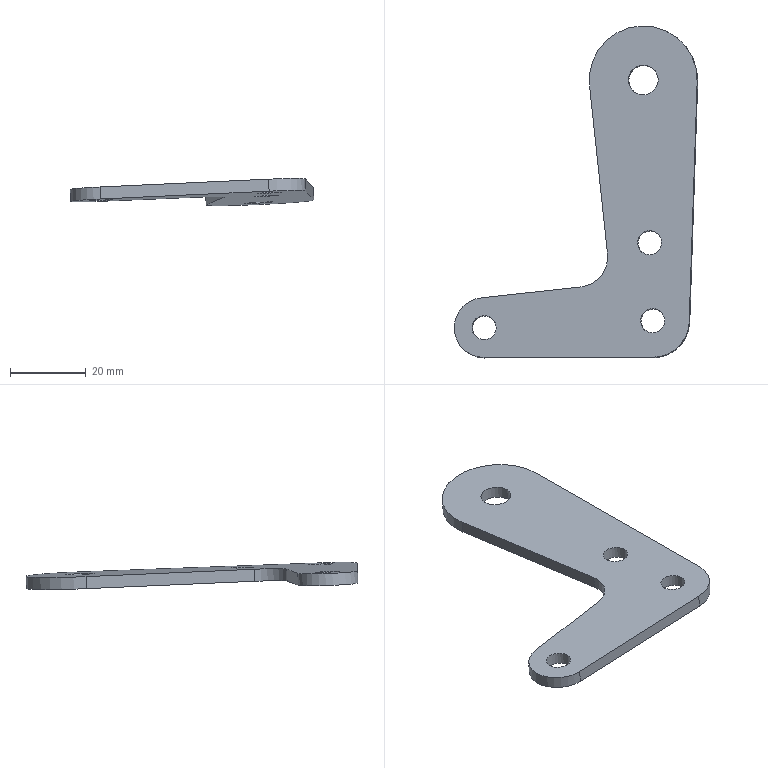Component | NX | RIOSTRA_B | 1 solid | 14 faces | box 64.12 x 87.41 x 7.19 mm | volume 8212 mm3 | cylinder 8 | plane 6 | commonest cylinder face diameters 6.35 x3 15.748 x2 28.448 x1 19.304 x1 7.874 x1
STEP:
#1=CARTESIAN_POINT('',(0.,0.,0.));
#2=DIRECTION('',(0.,0.,1.));
#3=DIRECTION('',(1.,0.,0.));
#4=AXIS2_PLACEMENT_3D('',#1,#2,#3);
#5=CARTESIAN_POINT('',(65.717,-19.594,13.451));
#6=VERTEX_POINT('',#5);
#7=CARTESIAN_POINT('',(21.35,-19.625,11.397));
#8=VERTEX_POINT('',#7);
#9=CARTESIAN_POINT('',(65.717,-19.594,13.451));
#10=DIRECTION('',(-0.9989,-0.0007017,-0.04625));
#11=VECTOR('',#10,1.);
#12=LINE('',#9,#11);
#13=CARTESIAN_POINT('',(65.57,-19.471,16.621));
#14=DIRECTION('',(-0.001095,-0.9992,0.0388));
#15=DIRECTION('',(0.9989,0.0007017,0.04625));
#16=AXIS2_PLACEMENT_3D('',#13,#14,#15);
#17=PLANE('',#16);
#18=CARTESIAN_POINT('',(-0.,-3.175));
#19=DIRECTION('',(-1.,-0.));
#20=VECTOR('',#19,1.);
#21=LINE('',#18,#20);
#22=(GEOMETRIC_REPRESENTATION_CONTEXT(2)PARAMETRIC_REPRESENTATION_CONTEXT()REPRESENTATION_CONTEXT('',''));
#23=DEFINITIONAL_REPRESENTATION('',(#21),#22);
#24=PCURVE('',#17,#23);
#25=CARTESIAN_POINT('',(21.359,-11.757,11.091));
#26=DIRECTION('',(0.04625,-0.03881,-0.9982));
#27=DIRECTION('',(0.03886,-0.9984,0.04062));
#28=AXIS2_PLACEMENT_3D('',#25,#26,#27);
#29=PLANE('',#28);
#30=CARTESIAN_POINT('',(9.644,-44.064));
#31=DIRECTION('',(-0.04,0.9992));
#32=VECTOR('',#31,1.);
#33=LINE('',#30,#32);
#34=(GEOMETRIC_REPRESENTATION_CONTEXT(2)PARAMETRIC_REPRESENTATION_CONTEXT()REPRESENTATION_CONTEXT('',''));
#35=DEFINITIONAL_REPRESENTATION('',(#33),#34);
#36=PCURVE('',#29,#35);
#37=SURFACE_CURVE('',#12,(#24,#36),.PCURVE_S1.);
#38=EDGE_CURVE('',#6,#8,#37,.T.);
#39=ORIENTED_EDGE('',*,*,#38,.F.);
#40=CARTESIAN_POINT('',(65.57,-19.471,16.621));
#41=VERTEX_POINT('',#40);
#42=CARTESIAN_POINT('',(65.57,-19.471,16.621));
#43=DIRECTION('',(0.04625,-0.03881,-0.9982));
#44=VECTOR('',#43,1.);
#45=LINE('',#42,#44);
#46=CARTESIAN_POINT('',(0.,0.));
#47=DIRECTION('',(0.,-1.));
#48=VECTOR('',#47,1.);
#49=LINE('',#46,#48);
#50=(GEOMETRIC_REPRESENTATION_CONTEXT(2)PARAMETRIC_REPRESENTATION_CONTEXT()REPRESENTATION_CONTEXT('',''));
#51=DEFINITIONAL_REPRESENTATION('',(#49),#50);
#52=PCURVE('',#17,#51);
#53=CARTESIAN_POINT('',(65.581,-9.826,16.246));
#54=DIRECTION('',(0.04625,-0.03881,-0.9982));
#55=DIRECTION('',(0.03886,-0.9984,0.04062));
#56=AXIS2_PLACEMENT_3D('',#53,#54,#55);
#57=CYLINDRICAL_SURFACE('',#56,9.652);
#58=CARTESIAN_POINT('',(6.323,-0.));
#59=DIRECTION('',(0.,1.));
#60=VECTOR('',#59,1.);
#61=LINE('',#58,#60);
#62=(GEOMETRIC_REPRESENTATION_CONTEXT(2)PARAMETRIC_REPRESENTATION_CONTEXT()REPRESENTATION_CONTEXT('',''));
#63=DEFINITIONAL_REPRESENTATION('',(#61),#62);
#64=PCURVE('',#57,#63);
#65=SURFACE_CURVE('',#45,(#52,#64),.PCURVE_S1.);
#66=EDGE_CURVE('',#41,#6,#65,.T.);
#67=ORIENTED_EDGE('',*,*,#66,.F.);
#68=CARTESIAN_POINT('',(21.203,-19.502,14.566));
#69=VERTEX_POINT('',#68);
#70=CARTESIAN_POINT('',(65.57,-19.471,16.621));
#71=DIRECTION('',(-0.9989,-0.0007017,-0.04625));
#72=VECTOR('',#71,1.);
#73=LINE('',#70,#72);
#74=CARTESIAN_POINT('',(0.,0.));
#75=DIRECTION('',(-1.,-0.));
#76=VECTOR('',#75,1.);
#77=LINE('',#74,#76);
#78=(GEOMETRIC_REPRESENTATION_CONTEXT(2)PARAMETRIC_REPRESENTATION_CONTEXT()REPRESENTATION_CONTEXT('',''));
#79=DEFINITIONAL_REPRESENTATION('',(#77),#78);
#80=PCURVE('',#17,#79);
#81=CARTESIAN_POINT('',(21.212,-11.634,14.261));
#82=DIRECTION('',(0.04625,-0.03881,-0.9982));
#83=DIRECTION('',(0.03886,-0.9984,0.04062));
#84=AXIS2_PLACEMENT_3D('',#81,#82,#83);
#85=PLANE('',#84);
#86=CARTESIAN_POINT('',(9.644,-44.064));
#87=DIRECTION('',(-0.04,0.9992));
#88=VECTOR('',#87,1.);
#89=LINE('',#86,#88);
#90=(GEOMETRIC_REPRESENTATION_CONTEXT(2)PARAMETRIC_REPRESENTATION_CONTEXT()REPRESENTATION_CONTEXT('',''));
#91=DEFINITIONAL_REPRESENTATION('',(#89),#90);
#92=PCURVE('',#85,#91);
#93=SURFACE_CURVE('',#73,(#80,#92),.PCURVE_S1.);
#94=EDGE_CURVE('',#41,#69,#93,.T.);
#95=ORIENTED_EDGE('',*,*,#94,.T.);
#96=CARTESIAN_POINT('',(21.203,-19.502,14.566));
#97=DIRECTION('',(0.04625,-0.03881,-0.9982));
#98=VECTOR('',#97,1.);
#99=LINE('',#96,#98);
#100=CARTESIAN_POINT('',(-44.414,-0.));
#101=DIRECTION('',(0.,-1.));
#102=VECTOR('',#101,1.);
#103=LINE('',#100,#102);
#104=(GEOMETRIC_REPRESENTATION_CONTEXT(2)PARAMETRIC_REPRESENTATION_CONTEXT()REPRESENTATION_CONTEXT('',''));
#105=DEFINITIONAL_REPRESENTATION('',(#103),#104);
#106=PCURVE('',#17,#105);
#107=CARTESIAN_POINT('',(21.212,-11.634,14.261));
#108=DIRECTION('',(0.04625,-0.03881,-0.9982));
#109=DIRECTION('',(0.03886,-0.9984,0.04062));
#110=AXIS2_PLACEMENT_3D('',#107,#108,#109);
#111=CYLINDRICAL_SURFACE('',#110,7.874);
#112=CARTESIAN_POINT('',(0.04001,0.));
#113=DIRECTION('',(-0.,1.));
#114=VECTOR('',#113,1.);
#115=LINE('',#112,#114);
#116=(GEOMETRIC_REPRESENTATION_CONTEXT(2)PARAMETRIC_REPRESENTATION_CONTEXT()REPRESENTATION_CONTEXT('',''));
#117=DEFINITIONAL_REPRESENTATION('',(#115),#116);
#118=PCURVE('',#111,#117);
#119=SURFACE_CURVE('',#99,(#106,#118),.PCURVE_S1.);
#120=EDGE_CURVE('',#69,#8,#119,.T.);
#121=ORIENTED_EDGE('',*,*,#120,.T.);
#122=EDGE_LOOP('',(#39,#67,#95,#121));
#123=FACE_BOUND('',#122,.T.);
#124=ADVANCED_FACE('',(#123),#17,.T.);
#125=CARTESIAN_POINT('',(20.739,-3.914,10.758));
#126=VERTEX_POINT('',#125);
#127=CARTESIAN_POINT('',(21.359,-11.757,11.091));
#128=DIRECTION('',(0.04625,-0.03881,-0.9982));
#129=DIRECTION('',(-0.03886,0.9984,-0.04062));
#130=AXIS2_PLACEMENT_3D('',#127,#128,#129);
#131=CIRCLE('',#130,7.874);
#132=CARTESIAN_POINT('',(-3.142,3.175));
#133=DIRECTION('',(1.,0.));
#134=VECTOR('',#133,1.);
#135=LINE('',#132,#134);
#136=(GEOMETRIC_REPRESENTATION_CONTEXT(2)PARAMETRIC_REPRESENTATION_CONTEXT()REPRESENTATION_CONTEXT('',''));
#137=DEFINITIONAL_REPRESENTATION('',(#135),#136);
#138=PCURVE('',#111,#137);
#139=CARTESIAN_POINT('',(0.,0.));
#140=DIRECTION('',(-1.,0.));
#141=AXIS2_PLACEMENT_2D('',#139,#140);
#142=CIRCLE('',#141,7.874);
#143=(GEOMETRIC_REPRESENTATION_CONTEXT(2)PARAMETRIC_REPRESENTATION_CONTEXT()REPRESENTATION_CONTEXT('',''));
#144=DEFINITIONAL_REPRESENTATION('',(#142),#143);
#145=PCURVE('',#29,#144);
#146=SURFACE_CURVE('',#131,(#138,#145),.PCURVE_S1.);
#147=EDGE_CURVE('',#8,#126,#146,.T.);
#148=ORIENTED_EDGE('',*,*,#147,.F.);
#149=ORIENTED_EDGE('',*,*,#120,.F.);
#150=CARTESIAN_POINT('',(20.592,-3.791,13.927));
#151=VERTEX_POINT('',#150);
#152=CARTESIAN_POINT('',(21.212,-11.634,14.261));
#153=DIRECTION('',(0.04625,-0.03881,-0.9982));
#154=DIRECTION('',(-0.03886,0.9984,-0.04062));
#155=AXIS2_PLACEMENT_3D('',#152,#153,#154);
#156=CIRCLE('',#155,7.874);
#157=CARTESIAN_POINT('',(-3.142,0.));
#158=DIRECTION('',(1.,0.));
#159=VECTOR('',#158,1.);
#160=LINE('',#157,#159);
#161=(GEOMETRIC_REPRESENTATION_CONTEXT(2)PARAMETRIC_REPRESENTATION_CONTEXT()REPRESENTATION_CONTEXT('',''));
#162=DEFINITIONAL_REPRESENTATION('',(#160),#161);
#163=PCURVE('',#111,#162);
#164=CARTESIAN_POINT('',(0.,0.));
#165=DIRECTION('',(-1.,0.));
#166=AXIS2_PLACEMENT_2D('',#164,#165);
#167=CIRCLE('',#166,7.874);
#168=(GEOMETRIC_REPRESENTATION_CONTEXT(2)PARAMETRIC_REPRESENTATION_CONTEXT()REPRESENTATION_CONTEXT('',''));
#169=DEFINITIONAL_REPRESENTATION('',(#167),#168);
#170=PCURVE('',#85,#169);
#171=SURFACE_CURVE('',#156,(#163,#170),.PCURVE_S1.);
#172=EDGE_CURVE('',#69,#151,#171,.T.);
#173=ORIENTED_EDGE('',*,*,#172,.T.);
#174=CARTESIAN_POINT('',(20.592,-3.791,13.927));
#175=DIRECTION('',(0.04625,-0.03881,-0.9982));
#176=VECTOR('',#175,1.);
#177=LINE('',#174,#176);
#178=CARTESIAN_POINT('',(3.102,-0.));
#179=DIRECTION('',(-0.,1.));
#180=VECTOR('',#179,1.);
#181=LINE('',#178,#180);
#182=(GEOMETRIC_REPRESENTATION_CONTEXT(2)PARAMETRIC_REPRESENTATION_CONTEXT()REPRESENTATION_CONTEXT('',''));
#183=DEFINITIONAL_REPRESENTATION('',(#181),#182);
#184=PCURVE('',#111,#183);
#185=CARTESIAN_POINT('',(20.592,-3.791,13.927));
#186=DIRECTION('',(-0.1072,0.9933,-0.04358));
#187=DIRECTION('',(-0.9932,-0.109,-0.04178));
#188=AXIS2_PLACEMENT_3D('',#185,#186,#187);
#189=PLANE('',#188);
#190=CARTESIAN_POINT('',(0.,0.));
#191=DIRECTION('',(-0.,-1.));
#192=VECTOR('',#191,1.);
#193=LINE('',#190,#192);
#194=(GEOMETRIC_REPRESENTATION_CONTEXT(2)PARAMETRIC_REPRESENTATION_CONTEXT()REPRESENTATION_CONTEXT('',''));
#195=DEFINITIONAL_REPRESENTATION('',(#193),#194);
#196=PCURVE('',#189,#195);
#197=SURFACE_CURVE('',#177,(#184,#196),.PCURVE_S1.);
#198=EDGE_CURVE('',#151,#126,#197,.T.);
#199=ORIENTED_EDGE('',*,*,#198,.T.);
#200=EDGE_LOOP('',(#148,#149,#173,#199));
#201=FACE_BOUND('',#200,.T.);
#202=ADVANCED_FACE('',(#201),#111,.T.);
#203=CARTESIAN_POINT('',(46.875,-1.047,11.857));
#204=VERTEX_POINT('',#203);
#205=CARTESIAN_POINT('',(20.739,-3.914,10.758));
#206=DIRECTION('',(0.9932,0.109,0.04178));
#207=VECTOR('',#206,1.);
#208=LINE('',#205,#207);
#209=CARTESIAN_POINT('',(0.,-3.175));
#210=DIRECTION('',(-1.,0.));
#211=VECTOR('',#210,1.);
#212=LINE('',#209,#211);
#213=(GEOMETRIC_REPRESENTATION_CONTEXT(2)PARAMETRIC_REPRESENTATION_CONTEXT()REPRESENTATION_CONTEXT('',''));
#214=DEFINITIONAL_REPRESENTATION('',(#212),#213);
#215=PCURVE('',#189,#214);
#216=CARTESIAN_POINT('',(-7.868,0.315));
#217=DIRECTION('',(-0.06851,-0.9977));
#218=VECTOR('',#217,1.);
#219=LINE('',#216,#218);
#220=(GEOMETRIC_REPRESENTATION_CONTEXT(2)PARAMETRIC_REPRESENTATION_CONTEXT()REPRESENTATION_CONTEXT('',''));
#221=DEFINITIONAL_REPRESENTATION('',(#219),#220);
#222=PCURVE('',#29,#221);
#223=SURFACE_CURVE('',#208,(#215,#222),.PCURVE_S1.);
#224=EDGE_CURVE('',#126,#204,#223,.T.);
#225=ORIENTED_EDGE('',*,*,#224,.F.);
#226=ORIENTED_EDGE('',*,*,#198,.F.);
#227=CARTESIAN_POINT('',(46.728,-0.9234,15.027));
#228=VERTEX_POINT('',#227);
#229=CARTESIAN_POINT('',(20.592,-3.791,13.927));
#230=DIRECTION('',(0.9932,0.109,0.04178));
#231=VECTOR('',#230,1.);
#232=LINE('',#229,#231);
#233=CARTESIAN_POINT('',(0.,0.));
#234=DIRECTION('',(-1.,0.));
#235=VECTOR('',#234,1.);
#236=LINE('',#233,#235);
#237=(GEOMETRIC_REPRESENTATION_CONTEXT(2)PARAMETRIC_REPRESENTATION_CONTEXT()REPRESENTATION_CONTEXT('',''));
#238=DEFINITIONAL_REPRESENTATION('',(#236),#237);
#239=PCURVE('',#189,#238);
#240=CARTESIAN_POINT('',(-7.868,0.315));
#241=DIRECTION('',(-0.06851,-0.9977));
#242=VECTOR('',#241,1.);
#243=LINE('',#240,#242);
#244=(GEOMETRIC_REPRESENTATION_CONTEXT(2)PARAMETRIC_REPRESENTATION_CONTEXT()REPRESENTATION_CONTEXT('',''));
#245=DEFINITIONAL_REPRESENTATION('',(#243),#244);
#246=PCURVE('',#85,#245);
#247=SURFACE_CURVE('',#232,(#239,#246),.PCURVE_S1.);
#248=EDGE_CURVE('',#151,#228,#247,.T.);
#249=ORIENTED_EDGE('',*,*,#248,.T.);
#250=CARTESIAN_POINT('',(46.728,-0.9234,15.027));
#251=DIRECTION('',(0.04625,-0.03881,-0.9982));
#252=VECTOR('',#251,1.);
#253=LINE('',#250,#252);
#254=CARTESIAN_POINT('',(-26.316,-0.));
#255=DIRECTION('',(-0.,-1.));
#256=VECTOR('',#255,1.);
#257=LINE('',#254,#256);
#258=(GEOMETRIC_REPRESENTATION_CONTEXT(2)PARAMETRIC_REPRESENTATION_CONTEXT()REPRESENTATION_CONTEXT('',''));
#259=DEFINITIONAL_REPRESENTATION('',(#257),#258);
#260=PCURVE('',#189,#259);
#261=CARTESIAN_POINT('',(45.885,6.898,14.683));
#262=DIRECTION('',(0.04625,-0.03881,-0.9982));
#263=DIRECTION('',(0.03886,-0.9984,0.04062));
#264=AXIS2_PLACEMENT_3D('',#261,#262,#263);
#265=CYLINDRICAL_SURFACE('',#264,7.874);
#266=CARTESIAN_POINT('',(6.215,0.));
#267=DIRECTION('',(0.,1.));
#268=VECTOR('',#267,1.);
#269=LINE('',#266,#268);
#270=(GEOMETRIC_REPRESENTATION_CONTEXT(2)PARAMETRIC_REPRESENTATION_CONTEXT()REPRESENTATION_CONTEXT('',''));
#271=DEFINITIONAL_REPRESENTATION('',(#269),#270);
#272=PCURVE('',#265,#271);
#273=SURFACE_CURVE('',#253,(#260,#272),.PCURVE_S1.);
#274=EDGE_CURVE('',#228,#204,#273,.T.);
#275=ORIENTED_EDGE('',*,*,#274,.T.);
#276=EDGE_LOOP('',(#225,#226,#249,#275));
#277=FACE_BOUND('',#276,.T.);
#278=ADVANCED_FACE('',(#277),#189,.T.);
#279=CARTESIAN_POINT('',(53.706,7.746,15.013));
#280=VERTEX_POINT('',#279);
#281=CARTESIAN_POINT('',(53.853,7.623,11.844));
#282=VERTEX_POINT('',#281);
#283=CARTESIAN_POINT('',(53.706,7.746,15.013));
#284=DIRECTION('',(0.04625,-0.03881,-0.9982));
#285=VECTOR('',#284,1.);
#286=LINE('',#283,#285);
#287=CARTESIAN_POINT('',(4.645,-0.));
#288=DIRECTION('',(0.,1.));
#289=VECTOR('',#288,1.);
#290=LINE('',#287,#289);
#291=(GEOMETRIC_REPRESENTATION_CONTEXT(2)PARAMETRIC_REPRESENTATION_CONTEXT()REPRESENTATION_CONTEXT('',''));
#292=DEFINITIONAL_REPRESENTATION('',(#290),#291);
#293=PCURVE('',#265,#292);
#294=CARTESIAN_POINT('',(53.706,7.746,15.013));
#295=DIRECTION('',(-0.9933,-0.1077,-0.04183));
#296=DIRECTION('',(0.1059,-0.9934,0.04353));
#297=AXIS2_PLACEMENT_3D('',#294,#295,#296);
#298=PLANE('',#297);
#299=CARTESIAN_POINT('',(-0.,0.));
#300=DIRECTION('',(0.,-1.));
#301=VECTOR('',#300,1.);
#302=LINE('',#299,#301);
#303=(GEOMETRIC_REPRESENTATION_CONTEXT(2)PARAMETRIC_REPRESENTATION_CONTEXT()REPRESENTATION_CONTEXT('',''));
#304=DEFINITIONAL_REPRESENTATION('',(#302),#303);
#305=PCURVE('',#298,#304);
#306=SURFACE_CURVE('',#286,(#293,#305),.PCURVE_S1.);
#307=EDGE_CURVE('',#280,#282,#306,.T.);
#308=ORIENTED_EDGE('',*,*,#307,.F.);
#309=CARTESIAN_POINT('',(45.885,6.898,14.683));
#310=DIRECTION('',(-0.04625,0.03881,0.9982));
#311=DIRECTION('',(-0.03886,0.9984,-0.04062));
#312=AXIS2_PLACEMENT_3D('',#309,#310,#311);
#313=CIRCLE('',#312,7.874);
#314=CARTESIAN_POINT('',(9.425,-0.));
#315=DIRECTION('',(-1.,0.));
#316=VECTOR('',#315,1.);
#317=LINE('',#314,#316);
#318=(GEOMETRIC_REPRESENTATION_CONTEXT(2)PARAMETRIC_REPRESENTATION_CONTEXT()REPRESENTATION_CONTEXT('',''));
#319=DEFINITIONAL_REPRESENTATION('',(#317),#318);
#320=PCURVE('',#265,#319);
#321=CARTESIAN_POINT('',(-25.4,-25.4));
#322=CARTESIAN_POINT('',(-25.4,-11.762));
#323=CARTESIAN_POINT('',(-13.589,-18.581));
#324=CARTESIAN_POINT('',(-1.778,-25.4));
#325=CARTESIAN_POINT('',(-13.589,-32.219));
#326=CARTESIAN_POINT('',(-25.4,-39.038));
#327=CARTESIAN_POINT('',(-25.4,-25.4));
#328=(BOUNDED_CURVE()B_SPLINE_CURVE(2,(#321,#322,#323,#324,#325,#326,#327),.UNSPECIFIED.,.T.,.F.)B_SPLINE_CURVE_WITH_KNOTS((1,2,2,2,2,1),(-2.094,0.,2.094,4.189,6.283,8.378),.UNSPECIFIED.)CURVE()GEOMETRIC_REPRESENTATION_ITEM()RATIONAL_B_SPLINE_CURVE((1.,0.5,1.,0.5,1.,0.5,1.))REPRESENTATION_ITEM(''));
#329=(GEOMETRIC_REPRESENTATION_CONTEXT(2)PARAMETRIC_REPRESENTATION_CONTEXT()REPRESENTATION_CONTEXT('',''));
#330=DEFINITIONAL_REPRESENTATION('',(#328),#329);
#331=PCURVE('',#85,#330);
#332=SURFACE_CURVE('',#313,(#320,#331),.PCURVE_S1.);
#333=EDGE_CURVE('',#228,#280,#332,.T.);
#334=ORIENTED_EDGE('',*,*,#333,.F.);
#335=ORIENTED_EDGE('',*,*,#274,.T.);
#336=CARTESIAN_POINT('',(46.031,6.775,11.514));
#337=DIRECTION('',(-0.04625,0.03881,0.9982));
#338=DIRECTION('',(-0.03886,0.9984,-0.04062));
#339=AXIS2_PLACEMENT_3D('',#336,#337,#338);
#340=CIRCLE('',#339,7.874);
#341=CARTESIAN_POINT('',(9.425,3.175));
#342=DIRECTION('',(-1.,0.));
#343=VECTOR('',#342,1.);
#344=LINE('',#341,#343);
#345=(GEOMETRIC_REPRESENTATION_CONTEXT(2)PARAMETRIC_REPRESENTATION_CONTEXT()REPRESENTATION_CONTEXT('',''));
#346=DEFINITIONAL_REPRESENTATION('',(#344),#345);
#347=PCURVE('',#265,#346);
#348=CARTESIAN_POINT('',(-25.4,-25.4));
#349=CARTESIAN_POINT('',(-25.4,-11.762));
#350=CARTESIAN_POINT('',(-13.589,-18.581));
#351=CARTESIAN_POINT('',(-1.778,-25.4));
#352=CARTESIAN_POINT('',(-13.589,-32.219));
#353=CARTESIAN_POINT('',(-25.4,-39.038));
#354=CARTESIAN_POINT('',(-25.4,-25.4));
#355=(BOUNDED_CURVE()B_SPLINE_CURVE(2,(#348,#349,#350,#351,#352,#353,#354),.UNSPECIFIED.,.T.,.F.)B_SPLINE_CURVE_WITH_KNOTS((1,2,2,2,2,1),(-2.094,0.,2.094,4.189,6.283,8.378),.UNSPECIFIED.)CURVE()GEOMETRIC_REPRESENTATION_ITEM()RATIONAL_B_SPLINE_CURVE((1.,0.5,1.,0.5,1.,0.5,1.))REPRESENTATION_ITEM(''));
#356=(GEOMETRIC_REPRESENTATION_CONTEXT(2)PARAMETRIC_REPRESENTATION_CONTEXT()REPRESENTATION_CONTEXT('',''));
#357=DEFINITIONAL_REPRESENTATION('',(#355),#356);
#358=PCURVE('',#29,#357);
#359=SURFACE_CURVE('',#340,(#347,#358),.PCURVE_S1.);
#360=EDGE_CURVE('',#204,#282,#359,.T.);
#361=ORIENTED_EDGE('',*,*,#360,.T.);
#362=EDGE_LOOP('',(#308,#334,#335,#361));
#363=FACE_BOUND('',#362,.F.);
#364=ADVANCED_FACE('',(#363),#265,.F.);
#365=CARTESIAN_POINT('',(49.138,51.851,9.906));
#366=VERTEX_POINT('',#365);
#367=CARTESIAN_POINT('',(53.853,7.623,11.844));
#368=DIRECTION('',(-0.1059,0.9934,-0.04353));
#369=VECTOR('',#368,1.);
#370=LINE('',#367,#369);
#371=CARTESIAN_POINT('',(-0.,-3.175));
#372=DIRECTION('',(-1.,0.));
#373=VECTOR('',#372,1.);
#374=LINE('',#371,#373);
#375=(GEOMETRIC_REPRESENTATION_CONTEXT(2)PARAMETRIC_REPRESENTATION_CONTEXT()REPRESENTATION_CONTEXT('',''));
#376=DEFINITIONAL_REPRESENTATION('',(#374),#375);
#377=PCURVE('',#298,#376);
#378=CARTESIAN_POINT('',(-18.055,-33.256));
#379=DIRECTION('',(-0.9977,0.06723));
#380=VECTOR('',#379,1.);
#381=LINE('',#378,#380);
#382=(GEOMETRIC_REPRESENTATION_CONTEXT(2)PARAMETRIC_REPRESENTATION_CONTEXT()REPRESENTATION_CONTEXT('',''));
#383=DEFINITIONAL_REPRESENTATION('',(#381),#382);
#384=PCURVE('',#29,#383);
#385=SURFACE_CURVE('',#370,(#377,#384),.PCURVE_S1.);
#386=EDGE_CURVE('',#282,#366,#385,.T.);
#387=ORIENTED_EDGE('',*,*,#386,.F.);
#388=ORIENTED_EDGE('',*,*,#307,.F.);
#389=CARTESIAN_POINT('',(48.992,51.974,13.075));
#390=VERTEX_POINT('',#389);
#391=CARTESIAN_POINT('',(53.706,7.746,15.013));
#392=DIRECTION('',(-0.1059,0.9934,-0.04353));
#393=VECTOR('',#392,1.);
#394=LINE('',#391,#393);
#395=CARTESIAN_POINT('',(0.,0.));
#396=DIRECTION('',(-1.,0.));
#397=VECTOR('',#396,1.);
#398=LINE('',#395,#397);
#399=(GEOMETRIC_REPRESENTATION_CONTEXT(2)PARAMETRIC_REPRESENTATION_CONTEXT()REPRESENTATION_CONTEXT('',''));
#400=DEFINITIONAL_REPRESENTATION('',(#398),#399);
#401=PCURVE('',#298,#400);
#402=CARTESIAN_POINT('',(-18.055,-33.256));
#403=DIRECTION('',(-0.9977,0.06723));
#404=VECTOR('',#403,1.);
#405=LINE('',#402,#404);
#406=(GEOMETRIC_REPRESENTATION_CONTEXT(2)PARAMETRIC_REPRESENTATION_CONTEXT()REPRESENTATION_CONTEXT('',''));
#407=DEFINITIONAL_REPRESENTATION('',(#405),#406);
#408=PCURVE('',#85,#407);
#409=SURFACE_CURVE('',#394,(#401,#408),.PCURVE_S1.);
#410=EDGE_CURVE('',#280,#390,#409,.T.);
#411=ORIENTED_EDGE('',*,*,#410,.T.);
#412=CARTESIAN_POINT('',(48.992,51.974,13.075));
#413=DIRECTION('',(0.04625,-0.03881,-0.9982));
#414=VECTOR('',#413,1.);
#415=LINE('',#412,#414);
#416=CARTESIAN_POINT('',(-44.521,-0.));
#417=DIRECTION('',(0.,-1.));
#418=VECTOR('',#417,1.);
#419=LINE('',#416,#418);
#420=(GEOMETRIC_REPRESENTATION_CONTEXT(2)PARAMETRIC_REPRESENTATION_CONTEXT()REPRESENTATION_CONTEXT('',''));
#421=DEFINITIONAL_REPRESENTATION('',(#419),#420);
#422=PCURVE('',#298,#421);
#423=CARTESIAN_POINT('',(63.113,53.574,13.667));
#424=DIRECTION('',(0.04625,-0.03881,-0.9982));
#425=DIRECTION('',(0.03886,-0.9984,0.04062));
#426=AXIS2_PLACEMENT_3D('',#423,#424,#425);
#427=CYLINDRICAL_SURFACE('',#426,14.224);
#428=CARTESIAN_POINT('',(1.499,0.));
#429=DIRECTION('',(0.,1.));
#430=VECTOR('',#429,1.);
#431=LINE('',#428,#430);
#432=(GEOMETRIC_REPRESENTATION_CONTEXT(2)PARAMETRIC_REPRESENTATION_CONTEXT()REPRESENTATION_CONTEXT('',''));
#433=DEFINITIONAL_REPRESENTATION('',(#431),#432);
#434=PCURVE('',#427,#433);
#435=SURFACE_CURVE('',#415,(#422,#434),.PCURVE_S1.);
#436=EDGE_CURVE('',#390,#366,#435,.T.);
#437=ORIENTED_EDGE('',*,*,#436,.T.);
#438=EDGE_LOOP('',(#387,#388,#411,#437));
#439=FACE_BOUND('',#438,.T.);
#440=ADVANCED_FACE('',(#439),#298,.T.);
#441=CARTESIAN_POINT('',(77.461,53.005,11.173));
#442=VERTEX_POINT('',#441);
#443=CARTESIAN_POINT('',(63.26,53.451,10.498));
#444=DIRECTION('',(0.04625,-0.03881,-0.9982));
#445=DIRECTION('',(-0.03886,0.9984,-0.04062));
#446=AXIS2_PLACEMENT_3D('',#443,#444,#445);
#447=CIRCLE('',#446,14.224);
#448=CARTESIAN_POINT('',(-3.142,3.175));
#449=DIRECTION('',(1.,0.));
#450=VECTOR('',#449,1.);
#451=LINE('',#448,#450);
#452=(GEOMETRIC_REPRESENTATION_CONTEXT(2)PARAMETRIC_REPRESENTATION_CONTEXT()REPRESENTATION_CONTEXT('',''));
#453=DEFINITIONAL_REPRESENTATION('',(#451),#452);
#454=PCURVE('',#427,#453);
#455=CARTESIAN_POINT('',(-63.5,-44.45));
#456=DIRECTION('',(-1.,-0.));
#457=AXIS2_PLACEMENT_2D('',#455,#456);
#458=CIRCLE('',#457,14.224);
#459=(GEOMETRIC_REPRESENTATION_CONTEXT(2)PARAMETRIC_REPRESENTATION_CONTEXT()REPRESENTATION_CONTEXT('',''));
#460=DEFINITIONAL_REPRESENTATION('',(#458),#459);
#461=PCURVE('',#29,#460);
#462=SURFACE_CURVE('',#447,(#454,#461),.PCURVE_S1.);
#463=EDGE_CURVE('',#366,#442,#462,.T.);
#464=ORIENTED_EDGE('',*,*,#463,.F.);
#465=ORIENTED_EDGE('',*,*,#436,.F.);
#466=CARTESIAN_POINT('',(77.314,53.128,14.342));
#467=VERTEX_POINT('',#466);
#468=CARTESIAN_POINT('',(63.113,53.574,13.667));
#469=DIRECTION('',(0.04625,-0.03881,-0.9982));
#470=DIRECTION('',(-0.03886,0.9984,-0.04062));
#471=AXIS2_PLACEMENT_3D('',#468,#469,#470);
#472=CIRCLE('',#471,14.224);
#473=CARTESIAN_POINT('',(-3.142,0.));
#474=DIRECTION('',(1.,0.));
#475=VECTOR('',#474,1.);
#476=LINE('',#473,#475);
#477=(GEOMETRIC_REPRESENTATION_CONTEXT(2)PARAMETRIC_REPRESENTATION_CONTEXT()REPRESENTATION_CONTEXT('',''));
#478=DEFINITIONAL_REPRESENTATION('',(#476),#477);
#479=PCURVE('',#427,#478);
#480=CARTESIAN_POINT('',(-63.5,-44.45));
#481=DIRECTION('',(-1.,-0.));
#482=AXIS2_PLACEMENT_2D('',#480,#481);
#483=CIRCLE('',#482,14.224);
#484=(GEOMETRIC_REPRESENTATION_CONTEXT(2)PARAMETRIC_REPRESENTATION_CONTEXT()REPRESENTATION_CONTEXT('',''));
#485=DEFINITIONAL_REPRESENTATION('',(#483),#484);
#486=PCURVE('',#85,#485);
#487=SURFACE_CURVE('',#472,(#479,#486),.PCURVE_S1.);
#488=EDGE_CURVE('',#390,#467,#487,.T.);
#489=ORIENTED_EDGE('',*,*,#488,.T.);
#490=CARTESIAN_POINT('',(77.314,53.128,14.342));
#491=DIRECTION('',(0.04625,-0.03881,-0.9982));
#492=VECTOR('',#491,1.);
#493=LINE('',#490,#492);
#494=CARTESIAN_POINT('',(4.784,-0.));
#495=DIRECTION('',(0.,1.));
#496=VECTOR('',#495,1.);
#497=LINE('',#494,#496);
#498=(GEOMETRIC_REPRESENTATION_CONTEXT(2)PARAMETRIC_REPRESENTATION_CONTEXT()REPRESENTATION_CONTEXT('',''));
#499=DEFINITIONAL_REPRESENTATION('',(#497),#498);
#500=PCURVE('',#427,#499);
#501=CARTESIAN_POINT('',(77.314,53.128,14.342));
#502=DIRECTION('',(0.9984,-0.03132,0.04747));
#503=DIRECTION('',(0.03311,0.9988,-0.03729));
#504=AXIS2_PLACEMENT_3D('',#501,#502,#503);
#505=PLANE('',#504);
#506=CARTESIAN_POINT('',(0.,0.));
#507=DIRECTION('',(-0.,-1.));
#508=VECTOR('',#507,1.);
#509=LINE('',#506,#508);
#510=(GEOMETRIC_REPRESENTATION_CONTEXT(2)PARAMETRIC_REPRESENTATION_CONTEXT()REPRESENTATION_CONTEXT('',''));
#511=DEFINITIONAL_REPRESENTATION('',(#509),#510);
#512=PCURVE('',#505,#511);
#513=SURFACE_CURVE('',#493,(#500,#512),.PCURVE_S1.);
#514=EDGE_CURVE('',#467,#442,#513,.T.);
#515=ORIENTED_EDGE('',*,*,#514,.T.);
#516=EDGE_LOOP('',(#464,#465,#489,#515));
#517=FACE_BOUND('',#516,.T.);
#518=ADVANCED_FACE('',(#517),#427,.T.);
#519=CARTESIAN_POINT('',(75.364,-10.251,13.535));
#520=VERTEX_POINT('',#519);
#521=CARTESIAN_POINT('',(77.461,53.005,11.173));
#522=DIRECTION('',(-0.03311,-0.9988,0.03729));
#523=VECTOR('',#522,1.);
#524=LINE('',#521,#523);
#525=CARTESIAN_POINT('',(-0.,-3.175));
#526=DIRECTION('',(-1.,0.));
#527=VECTOR('',#526,1.);
#528=LINE('',#525,#527);
#529=(GEOMETRIC_REPRESENTATION_CONTEXT(2)PARAMETRIC_REPRESENTATION_CONTEXT()REPRESENTATION_CONTEXT('',''));
#530=DEFINITIONAL_REPRESENTATION('',(#528),#529);
#531=PCURVE('',#505,#530);
#532=CARTESIAN_POINT('',(-62.476,-58.637));
#533=DIRECTION('',(0.9974,0.072));
#534=VECTOR('',#533,1.);
#535=LINE('',#532,#534);
#536=(GEOMETRIC_REPRESENTATION_CONTEXT(2)PARAMETRIC_REPRESENTATION_CONTEXT()REPRESENTATION_CONTEXT('',''));
#537=DEFINITIONAL_REPRESENTATION('',(#535),#536);
#538=PCURVE('',#29,#537);
#539=SURFACE_CURVE('',#524,(#531,#538),.PCURVE_S1.);
#540=EDGE_CURVE('',#442,#520,#539,.T.);
#541=ORIENTED_EDGE('',*,*,#540,.F.);
#542=ORIENTED_EDGE('',*,*,#514,.F.);
#543=CARTESIAN_POINT('',(75.217,-10.128,16.704));
#544=VERTEX_POINT('',#543);
#545=CARTESIAN_POINT('',(77.314,53.128,14.342));
#546=DIRECTION('',(-0.03311,-0.9988,0.03729));
#547=VECTOR('',#546,1.);
#548=LINE('',#545,#547);
#549=CARTESIAN_POINT('',(0.,0.));
#550=DIRECTION('',(-1.,0.));
#551=VECTOR('',#550,1.);
#552=LINE('',#549,#551);
#553=(GEOMETRIC_REPRESENTATION_CONTEXT(2)PARAMETRIC_REPRESENTATION_CONTEXT()REPRESENTATION_CONTEXT('',''));
#554=DEFINITIONAL_REPRESENTATION('',(#552),#553);
#555=PCURVE('',#505,#554);
#556=CARTESIAN_POINT('',(-62.476,-58.637));
#557=DIRECTION('',(0.9974,0.072));
#558=VECTOR('',#557,1.);
#559=LINE('',#556,#558);
#560=(GEOMETRIC_REPRESENTATION_CONTEXT(2)PARAMETRIC_REPRESENTATION_CONTEXT()REPRESENTATION_CONTEXT('',''));
#561=DEFINITIONAL_REPRESENTATION('',(#559),#560);
#562=PCURVE('',#85,#561);
#563=SURFACE_CURVE('',#548,(#555,#562),.PCURVE_S1.);
#564=EDGE_CURVE('',#467,#544,#563,.T.);
#565=ORIENTED_EDGE('',*,*,#564,.T.);
#566=CARTESIAN_POINT('',(75.217,-10.128,16.704));
#567=DIRECTION('',(0.04625,-0.03881,-0.9982));
#568=VECTOR('',#567,1.);
#569=LINE('',#566,#568);
#570=CARTESIAN_POINT('',(-63.335,-0.));
#571=DIRECTION('',(-0.,-1.));
#572=VECTOR('',#571,1.);
#573=LINE('',#570,#572);
#574=(GEOMETRIC_REPRESENTATION_CONTEXT(2)PARAMETRIC_REPRESENTATION_CONTEXT()REPRESENTATION_CONTEXT('',''));
#575=DEFINITIONAL_REPRESENTATION('',(#573),#574);
#576=PCURVE('',#505,#575);
#577=CARTESIAN_POINT('',(4.784,0.));
#578=DIRECTION('',(0.,1.));
#579=VECTOR('',#578,1.);
#580=LINE('',#577,#579);
#581=(GEOMETRIC_REPRESENTATION_CONTEXT(2)PARAMETRIC_REPRESENTATION_CONTEXT()REPRESENTATION_CONTEXT('',''));
#582=DEFINITIONAL_REPRESENTATION('',(#580),#581);
#583=PCURVE('',#57,#582);
#584=SURFACE_CURVE('',#569,(#576,#583),.PCURVE_S1.);
#585=EDGE_CURVE('',#544,#520,#584,.T.);
#586=ORIENTED_EDGE('',*,*,#585,.T.);
#587=EDGE_LOOP('',(#541,#542,#565,#586));
#588=FACE_BOUND('',#587,.T.);
#589=ADVANCED_FACE('',(#588),#505,.T.);
#590=CARTESIAN_POINT('',(21.089,-8.464,14.132));
#591=VERTEX_POINT('',#590);
#592=CARTESIAN_POINT('',(21.212,-11.634,14.261));
#593=DIRECTION('',(0.04625,-0.03881,-0.9982));
#594=DIRECTION('',(-0.03886,0.9984,-0.04062));
#595=AXIS2_PLACEMENT_3D('',#592,#593,#594);
#596=CIRCLE('',#595,3.175);
#597=CARTESIAN_POINT('',(21.212,-11.634,14.261));
#598=DIRECTION('',(0.04625,-0.03881,-0.9982));
#599=DIRECTION('',(0.03886,-0.9984,0.04062));
#600=AXIS2_PLACEMENT_3D('',#597,#598,#599);
#601=CYLINDRICAL_SURFACE('',#600,3.175);
#602=CARTESIAN_POINT('',(3.142,0.));
#603=DIRECTION('',(1.,0.));
#604=VECTOR('',#603,1.);
#605=LINE('',#602,#604);
#606=(GEOMETRIC_REPRESENTATION_CONTEXT(2)PARAMETRIC_REPRESENTATION_CONTEXT()REPRESENTATION_CONTEXT('',''));
#607=DEFINITIONAL_REPRESENTATION('',(#605),#606);
#608=PCURVE('',#601,#607);
#609=CARTESIAN_POINT('',(0.,0.));
#610=DIRECTION('',(-1.,-0.));
#611=AXIS2_PLACEMENT_2D('',#609,#610);
#612=CIRCLE('',#611,3.175);
#613=(GEOMETRIC_REPRESENTATION_CONTEXT(2)PARAMETRIC_REPRESENTATION_CONTEXT()REPRESENTATION_CONTEXT('',''));
#614=DEFINITIONAL_REPRESENTATION('',(#612),#613);
#615=PCURVE('',#85,#614);
#616=SURFACE_CURVE('',#596,(#608,#615),.PCURVE_S1.);
#617=EDGE_CURVE('',#591,#591,#616,.T.);
#618=ORIENTED_EDGE('',*,*,#617,.T.);
#619=CARTESIAN_POINT('',(21.235,-8.587,10.963));
#620=VERTEX_POINT('',#619);
#621=CARTESIAN_POINT('',(21.089,-8.464,14.132));
#622=CARTESIAN_POINT('',(21.235,-8.587,10.963));
#623=B_SPLINE_CURVE_WITH_KNOTS('',1,(#621,#622),.UNSPECIFIED.,.F.,.F.,(2,2),(0.,3.175),.PIECEWISE_BEZIER_KNOTS.);
#624=CARTESIAN_POINT('',(9.425,0.));
#625=DIRECTION('',(0.,1.));
#626=VECTOR('',#625,1.);
#627=LINE('',#624,#626);
#628=(GEOMETRIC_REPRESENTATION_CONTEXT(2)PARAMETRIC_REPRESENTATION_CONTEXT()REPRESENTATION_CONTEXT('',''));
#629=DEFINITIONAL_REPRESENTATION('',(#627),#628);
#630=PCURVE('',#601,#629);
#631=CARTESIAN_POINT('',(3.142,0.));
#632=DIRECTION('',(0.,1.));
#633=VECTOR('',#632,1.);
#634=LINE('',#631,#633);
#635=(GEOMETRIC_REPRESENTATION_CONTEXT(2)PARAMETRIC_REPRESENTATION_CONTEXT()REPRESENTATION_CONTEXT('',''));
#636=DEFINITIONAL_REPRESENTATION('',(#634),#635);
#637=PCURVE('',#601,#636);
#638=SEAM_CURVE('',#623,(#630,#637),.PCURVE_S1.);
#639=EDGE_CURVE('',#591,#620,#638,.T.);
#640=ORIENTED_EDGE('',*,*,#639,.T.);
#641=CARTESIAN_POINT('',(21.359,-11.757,11.091));
#642=DIRECTION('',(0.04625,-0.03881,-0.9982));
#643=DIRECTION('',(-0.03886,0.9984,-0.04062));
#644=AXIS2_PLACEMENT_3D('',#641,#642,#643);
#645=CIRCLE('',#644,3.175);
#646=CARTESIAN_POINT('',(3.142,3.175));
#647=DIRECTION('',(1.,0.));
#648=VECTOR('',#647,1.);
#649=LINE('',#646,#648);
#650=(GEOMETRIC_REPRESENTATION_CONTEXT(2)PARAMETRIC_REPRESENTATION_CONTEXT()REPRESENTATION_CONTEXT('',''));
#651=DEFINITIONAL_REPRESENTATION('',(#649),#650);
#652=PCURVE('',#601,#651);
#653=CARTESIAN_POINT('',(0.,0.));
#654=DIRECTION('',(-1.,-0.));
#655=AXIS2_PLACEMENT_2D('',#653,#654);
#656=CIRCLE('',#655,3.175);
#657=(GEOMETRIC_REPRESENTATION_CONTEXT(2)PARAMETRIC_REPRESENTATION_CONTEXT()REPRESENTATION_CONTEXT('',''));
#658=DEFINITIONAL_REPRESENTATION('',(#656),#657);
#659=PCURVE('',#29,#658);
#660=SURFACE_CURVE('',#645,(#652,#659),.PCURVE_S1.);
#661=EDGE_CURVE('',#620,#620,#660,.T.);
#662=ORIENTED_EDGE('',*,*,#661,.F.);
#663=ORIENTED_EDGE('',*,*,#639,.F.);
#664=EDGE_LOOP('',(#618,#640,#662,#663));
#665=FACE_BOUND('',#664,.F.);
#666=ADVANCED_FACE('',(#665),#601,.F.);
#667=CARTESIAN_POINT('',(65.457,-6.656,16.117));
#668=VERTEX_POINT('',#667);
#669=CARTESIAN_POINT('',(65.581,-9.826,16.246));
#670=DIRECTION('',(0.04625,-0.03881,-0.9982));
#671=DIRECTION('',(-0.03886,0.9984,-0.04062));
#672=AXIS2_PLACEMENT_3D('',#669,#670,#671);
#673=CIRCLE('',#672,3.175);
#674=CARTESIAN_POINT('',(65.581,-9.826,16.246));
#675=DIRECTION('',(0.04625,-0.03881,-0.9982));
#676=DIRECTION('',(0.03886,-0.9984,0.04062));
#677=AXIS2_PLACEMENT_3D('',#674,#675,#676);
#678=CYLINDRICAL_SURFACE('',#677,3.175);
#679=CARTESIAN_POINT('',(3.142,0.));
#680=DIRECTION('',(1.,0.));
#681=VECTOR('',#680,1.);
#682=LINE('',#679,#681);
#683=(GEOMETRIC_REPRESENTATION_CONTEXT(2)PARAMETRIC_REPRESENTATION_CONTEXT()REPRESENTATION_CONTEXT('',''));
#684=DEFINITIONAL_REPRESENTATION('',(#682),#683);
#685=PCURVE('',#678,#684);
#686=CARTESIAN_POINT('',(-0.,-44.45));
#687=DIRECTION('',(-1.,0.));
#688=AXIS2_PLACEMENT_2D('',#686,#687);
#689=CIRCLE('',#688,3.175);
#690=(GEOMETRIC_REPRESENTATION_CONTEXT(2)PARAMETRIC_REPRESENTATION_CONTEXT()REPRESENTATION_CONTEXT('',''));
#691=DEFINITIONAL_REPRESENTATION('',(#689),#690);
#692=PCURVE('',#85,#691);
#693=SURFACE_CURVE('',#673,(#685,#692),.PCURVE_S1.);
#694=EDGE_CURVE('',#668,#668,#693,.T.);
#695=ORIENTED_EDGE('',*,*,#694,.T.);
#696=CARTESIAN_POINT('',(65.604,-6.779,12.948));
#697=VERTEX_POINT('',#696);
#698=CARTESIAN_POINT('',(65.457,-6.656,16.117));
#699=CARTESIAN_POINT('',(65.604,-6.779,12.948));
#700=B_SPLINE_CURVE_WITH_KNOTS('',1,(#698,#699),.UNSPECIFIED.,.F.,.F.,(2,2),(0.,3.175),.PIECEWISE_BEZIER_KNOTS.);
#701=CARTESIAN_POINT('',(9.425,0.));
#702=DIRECTION('',(0.,1.));
#703=VECTOR('',#702,1.);
#704=LINE('',#701,#703);
#705=(GEOMETRIC_REPRESENTATION_CONTEXT(2)PARAMETRIC_REPRESENTATION_CONTEXT()REPRESENTATION_CONTEXT('',''));
#706=DEFINITIONAL_REPRESENTATION('',(#704),#705);
#707=PCURVE('',#678,#706);
#708=CARTESIAN_POINT('',(3.142,0.));
#709=DIRECTION('',(0.,1.));
#710=VECTOR('',#709,1.);
#711=LINE('',#708,#710);
#712=(GEOMETRIC_REPRESENTATION_CONTEXT(2)PARAMETRIC_REPRESENTATION_CONTEXT()REPRESENTATION_CONTEXT('',''));
#713=DEFINITIONAL_REPRESENTATION('',(#711),#712);
#714=PCURVE('',#678,#713);
#715=SEAM_CURVE('',#700,(#707,#714),.PCURVE_S1.);
#716=EDGE_CURVE('',#668,#697,#715,.T.);
#717=ORIENTED_EDGE('',*,*,#716,.T.);
#718=CARTESIAN_POINT('',(65.728,-9.949,13.077));
#719=DIRECTION('',(0.04625,-0.03881,-0.9982));
#720=DIRECTION('',(-0.03886,0.9984,-0.04062));
#721=AXIS2_PLACEMENT_3D('',#718,#719,#720);
#722=CIRCLE('',#721,3.175);
#723=CARTESIAN_POINT('',(3.142,3.175));
#724=DIRECTION('',(1.,0.));
#725=VECTOR('',#724,1.);
#726=LINE('',#723,#725);
#727=(GEOMETRIC_REPRESENTATION_CONTEXT(2)PARAMETRIC_REPRESENTATION_CONTEXT()REPRESENTATION_CONTEXT('',''));
#728=DEFINITIONAL_REPRESENTATION('',(#726),#727);
#729=PCURVE('',#678,#728);
#730=CARTESIAN_POINT('',(-0.,-44.45));
#731=DIRECTION('',(-1.,0.));
#732=AXIS2_PLACEMENT_2D('',#730,#731);
#733=CIRCLE('',#732,3.175);
#734=(GEOMETRIC_REPRESENTATION_CONTEXT(2)PARAMETRIC_REPRESENTATION_CONTEXT()REPRESENTATION_CONTEXT('',''));
#735=DEFINITIONAL_REPRESENTATION('',(#733),#734);
#736=PCURVE('',#29,#735);
#737=SURFACE_CURVE('',#722,(#729,#736),.PCURVE_S1.);
#738=EDGE_CURVE('',#697,#697,#737,.T.);
#739=ORIENTED_EDGE('',*,*,#738,.F.);
#740=ORIENTED_EDGE('',*,*,#716,.F.);
#741=EDGE_LOOP('',(#695,#717,#739,#740));
#742=FACE_BOUND('',#741,.F.);
#743=ADVANCED_FACE('',(#742),#678,.F.);
#744=CARTESIAN_POINT('',(64.658,13.886,15.281));
#745=VERTEX_POINT('',#744);
#746=CARTESIAN_POINT('',(64.781,10.716,15.41));
#747=DIRECTION('',(0.04625,-0.03881,-0.9982));
#748=DIRECTION('',(-0.03886,0.9984,-0.04062));
#749=AXIS2_PLACEMENT_3D('',#746,#747,#748);
#750=CIRCLE('',#749,3.175);
#751=CARTESIAN_POINT('',(64.781,10.716,15.41));
#752=DIRECTION('',(0.04625,-0.03881,-0.9982));
#753=DIRECTION('',(0.03886,-0.9984,0.04062));
#754=AXIS2_PLACEMENT_3D('',#751,#752,#753);
#755=CYLINDRICAL_SURFACE('',#754,3.175);
#756=CARTESIAN_POINT('',(3.142,-0.));
#757=DIRECTION('',(1.,0.));
#758=VECTOR('',#757,1.);
#759=LINE('',#756,#758);
#760=(GEOMETRIC_REPRESENTATION_CONTEXT(2)PARAMETRIC_REPRESENTATION_CONTEXT()REPRESENTATION_CONTEXT('',''));
#761=DEFINITIONAL_REPRESENTATION('',(#759),#760);
#762=PCURVE('',#755,#761);
#763=CARTESIAN_POINT('',(-20.574,-44.45));
#764=DIRECTION('',(-1.,0.));
#765=AXIS2_PLACEMENT_2D('',#763,#764);
#766=CIRCLE('',#765,3.175);
#767=(GEOMETRIC_REPRESENTATION_CONTEXT(2)PARAMETRIC_REPRESENTATION_CONTEXT()REPRESENTATION_CONTEXT('',''));
#768=DEFINITIONAL_REPRESENTATION('',(#766),#767);
#769=PCURVE('',#85,#768);
#770=SURFACE_CURVE('',#750,(#762,#769),.PCURVE_S1.);
#771=EDGE_CURVE('',#745,#745,#770,.T.);
#772=ORIENTED_EDGE('',*,*,#771,.T.);
#773=CARTESIAN_POINT('',(64.805,13.762,12.112));
#774=VERTEX_POINT('',#773);
#775=CARTESIAN_POINT('',(64.658,13.886,15.281));
#776=CARTESIAN_POINT('',(64.805,13.762,12.112));
#777=B_SPLINE_CURVE_WITH_KNOTS('',1,(#775,#776),.UNSPECIFIED.,.F.,.F.,(2,2),(-0.,3.175),.PIECEWISE_BEZIER_KNOTS.);
#778=CARTESIAN_POINT('',(9.425,0.));
#779=DIRECTION('',(0.,1.));
#780=VECTOR('',#779,1.);
#781=LINE('',#778,#780);
#782=(GEOMETRIC_REPRESENTATION_CONTEXT(2)PARAMETRIC_REPRESENTATION_CONTEXT()REPRESENTATION_CONTEXT('',''));
#783=DEFINITIONAL_REPRESENTATION('',(#781),#782);
#784=PCURVE('',#755,#783);
#785=CARTESIAN_POINT('',(3.142,0.));
#786=DIRECTION('',(0.,1.));
#787=VECTOR('',#786,1.);
#788=LINE('',#785,#787);
#789=(GEOMETRIC_REPRESENTATION_CONTEXT(2)PARAMETRIC_REPRESENTATION_CONTEXT()REPRESENTATION_CONTEXT('',''));
#790=DEFINITIONAL_REPRESENTATION('',(#788),#789);
#791=PCURVE('',#755,#790);
#792=SEAM_CURVE('',#777,(#784,#791),.PCURVE_S1.);
#793=EDGE_CURVE('',#745,#774,#792,.T.);
#794=ORIENTED_EDGE('',*,*,#793,.T.);
#795=CARTESIAN_POINT('',(64.928,10.592,12.241));
#796=DIRECTION('',(0.04625,-0.03881,-0.9982));
#797=DIRECTION('',(-0.03886,0.9984,-0.04062));
#798=AXIS2_PLACEMENT_3D('',#795,#796,#797);
#799=CIRCLE('',#798,3.175);
#800=CARTESIAN_POINT('',(3.142,3.175));
#801=DIRECTION('',(1.,0.));
#802=VECTOR('',#801,1.);
#803=LINE('',#800,#802);
#804=(GEOMETRIC_REPRESENTATION_CONTEXT(2)PARAMETRIC_REPRESENTATION_CONTEXT()REPRESENTATION_CONTEXT('',''));
#805=DEFINITIONAL_REPRESENTATION('',(#803),#804);
#806=PCURVE('',#755,#805);
#807=CARTESIAN_POINT('',(-20.574,-44.45));
#808=DIRECTION('',(-1.,0.));
#809=AXIS2_PLACEMENT_2D('',#807,#808);
#810=CIRCLE('',#809,3.175);
#811=(GEOMETRIC_REPRESENTATION_CONTEXT(2)PARAMETRIC_REPRESENTATION_CONTEXT()REPRESENTATION_CONTEXT('',''));
#812=DEFINITIONAL_REPRESENTATION('',(#810),#811);
#813=PCURVE('',#29,#812);
#814=SURFACE_CURVE('',#799,(#806,#813),.PCURVE_S1.);
#815=EDGE_CURVE('',#774,#774,#814,.T.);
#816=ORIENTED_EDGE('',*,*,#815,.F.);
#817=ORIENTED_EDGE('',*,*,#793,.F.);
#818=EDGE_LOOP('',(#772,#794,#816,#817));
#819=FACE_BOUND('',#818,.F.);
#820=ADVANCED_FACE('',(#819),#755,.F.);
#821=CARTESIAN_POINT('',(65.728,-9.949,13.077));
#822=DIRECTION('',(0.04625,-0.03881,-0.9982));
#823=DIRECTION('',(-0.03886,0.9984,-0.04062));
#824=AXIS2_PLACEMENT_3D('',#821,#822,#823);
#825=CIRCLE('',#824,9.652);
#826=CARTESIAN_POINT('',(3.142,3.175));
#827=DIRECTION('',(1.,0.));
#828=VECTOR('',#827,1.);
#829=LINE('',#826,#828);
#830=(GEOMETRIC_REPRESENTATION_CONTEXT(2)PARAMETRIC_REPRESENTATION_CONTEXT()REPRESENTATION_CONTEXT('',''));
#831=DEFINITIONAL_REPRESENTATION('',(#829),#830);
#832=PCURVE('',#57,#831);
#833=CARTESIAN_POINT('',(-0.,-44.45));
#834=DIRECTION('',(-1.,0.));
#835=AXIS2_PLACEMENT_2D('',#833,#834);
#836=CIRCLE('',#835,9.652);
#837=(GEOMETRIC_REPRESENTATION_CONTEXT(2)PARAMETRIC_REPRESENTATION_CONTEXT()REPRESENTATION_CONTEXT('',''));
#838=DEFINITIONAL_REPRESENTATION('',(#836),#837);
#839=PCURVE('',#29,#838);
#840=SURFACE_CURVE('',#825,(#832,#839),.PCURVE_S1.);
#841=EDGE_CURVE('',#520,#6,#840,.T.);
#842=ORIENTED_EDGE('',*,*,#841,.F.);
#843=ORIENTED_EDGE('',*,*,#585,.F.);
#844=CARTESIAN_POINT('',(65.581,-9.826,16.246));
#845=DIRECTION('',(0.04625,-0.03881,-0.9982));
#846=DIRECTION('',(-0.03886,0.9984,-0.04062));
#847=AXIS2_PLACEMENT_3D('',#844,#845,#846);
#848=CIRCLE('',#847,9.652);
#849=CARTESIAN_POINT('',(3.142,0.));
#850=DIRECTION('',(1.,0.));
#851=VECTOR('',#850,1.);
#852=LINE('',#849,#851);
#853=(GEOMETRIC_REPRESENTATION_CONTEXT(2)PARAMETRIC_REPRESENTATION_CONTEXT()REPRESENTATION_CONTEXT('',''));
#854=DEFINITIONAL_REPRESENTATION('',(#852),#853);
#855=PCURVE('',#57,#854);
#856=CARTESIAN_POINT('',(-0.,-44.45));
#857=DIRECTION('',(-1.,0.));
#858=AXIS2_PLACEMENT_2D('',#856,#857);
#859=CIRCLE('',#858,9.652);
#860=(GEOMETRIC_REPRESENTATION_CONTEXT(2)PARAMETRIC_REPRESENTATION_CONTEXT()REPRESENTATION_CONTEXT('',''));
#861=DEFINITIONAL_REPRESENTATION('',(#859),#860);
#862=PCURVE('',#85,#861);
#863=SURFACE_CURVE('',#848,(#855,#862),.PCURVE_S1.);
#864=EDGE_CURVE('',#544,#41,#863,.T.);
#865=ORIENTED_EDGE('',*,*,#864,.T.);
#866=ORIENTED_EDGE('',*,*,#66,.T.);
#867=EDGE_LOOP('',(#842,#843,#865,#866));
#868=FACE_BOUND('',#867,.T.);
#869=ADVANCED_FACE('',(#868),#57,.T.);
#870=CARTESIAN_POINT('',(62.96,57.505,13.507));
#871=VERTEX_POINT('',#870);
#872=CARTESIAN_POINT('',(63.113,53.574,13.667));
#873=DIRECTION('',(0.04625,-0.03881,-0.9982));
#874=DIRECTION('',(-0.03886,0.9984,-0.04062));
#875=AXIS2_PLACEMENT_3D('',#872,#873,#874);
#876=CIRCLE('',#875,3.937);
#877=CARTESIAN_POINT('',(63.113,53.574,13.667));
#878=DIRECTION('',(0.04625,-0.03881,-0.9982));
#879=DIRECTION('',(0.03886,-0.9984,0.04062));
#880=AXIS2_PLACEMENT_3D('',#877,#878,#879);
#881=CYLINDRICAL_SURFACE('',#880,3.937);
#882=CARTESIAN_POINT('',(3.142,0.));
#883=DIRECTION('',(1.,0.));
#884=VECTOR('',#883,1.);
#885=LINE('',#882,#884);
#886=(GEOMETRIC_REPRESENTATION_CONTEXT(2)PARAMETRIC_REPRESENTATION_CONTEXT()REPRESENTATION_CONTEXT('',''));
#887=DEFINITIONAL_REPRESENTATION('',(#885),#886);
#888=PCURVE('',#881,#887);
#889=CARTESIAN_POINT('',(-63.5,-44.45));
#890=DIRECTION('',(-1.,-0.));
#891=AXIS2_PLACEMENT_2D('',#889,#890);
#892=CIRCLE('',#891,3.937);
#893=(GEOMETRIC_REPRESENTATION_CONTEXT(2)PARAMETRIC_REPRESENTATION_CONTEXT()REPRESENTATION_CONTEXT('',''));
#894=DEFINITIONAL_REPRESENTATION('',(#892),#893);
#895=PCURVE('',#85,#894);
#896=SURFACE_CURVE('',#876,(#888,#895),.PCURVE_S1.);
#897=EDGE_CURVE('',#871,#871,#896,.T.);
#898=ORIENTED_EDGE('',*,*,#897,.T.);
#899=CARTESIAN_POINT('',(63.107,57.381,10.338));
#900=VERTEX_POINT('',#899);
#901=CARTESIAN_POINT('',(62.96,57.505,13.507));
#902=CARTESIAN_POINT('',(63.107,57.381,10.338));
#903=B_SPLINE_CURVE_WITH_KNOTS('',1,(#901,#902),.UNSPECIFIED.,.F.,.F.,(2,2),(0.,3.175),.PIECEWISE_BEZIER_KNOTS.);
#904=CARTESIAN_POINT('',(9.425,0.));
#905=DIRECTION('',(0.,1.));
#906=VECTOR('',#905,1.);
#907=LINE('',#904,#906);
#908=(GEOMETRIC_REPRESENTATION_CONTEXT(2)PARAMETRIC_REPRESENTATION_CONTEXT()REPRESENTATION_CONTEXT('',''));
#909=DEFINITIONAL_REPRESENTATION('',(#907),#908);
#910=PCURVE('',#881,#909);
#911=CARTESIAN_POINT('',(3.142,0.));
#912=DIRECTION('',(0.,1.));
#913=VECTOR('',#912,1.);
#914=LINE('',#911,#913);
#915=(GEOMETRIC_REPRESENTATION_CONTEXT(2)PARAMETRIC_REPRESENTATION_CONTEXT()REPRESENTATION_CONTEXT('',''));
#916=DEFINITIONAL_REPRESENTATION('',(#914),#915);
#917=PCURVE('',#881,#916);
#918=SEAM_CURVE('',#903,(#910,#917),.PCURVE_S1.);
#919=EDGE_CURVE('',#871,#900,#918,.T.);
#920=ORIENTED_EDGE('',*,*,#919,.T.);
#921=CARTESIAN_POINT('',(63.26,53.451,10.498));
#922=DIRECTION('',(0.04625,-0.03881,-0.9982));
#923=DIRECTION('',(-0.03886,0.9984,-0.04062));
#924=AXIS2_PLACEMENT_3D('',#921,#922,#923);
#925=CIRCLE('',#924,3.937);
#926=CARTESIAN_POINT('',(3.142,3.175));
#927=DIRECTION('',(1.,0.));
#928=VECTOR('',#927,1.);
#929=LINE('',#926,#928);
#930=(GEOMETRIC_REPRESENTATION_CONTEXT(2)PARAMETRIC_REPRESENTATION_CONTEXT()REPRESENTATION_CONTEXT('',''));
#931=DEFINITIONAL_REPRESENTATION('',(#929),#930);
#932=PCURVE('',#881,#931);
#933=CARTESIAN_POINT('',(-63.5,-44.45));
#934=DIRECTION('',(-1.,-0.));
#935=AXIS2_PLACEMENT_2D('',#933,#934);
#936=CIRCLE('',#935,3.937);
#937=(GEOMETRIC_REPRESENTATION_CONTEXT(2)PARAMETRIC_REPRESENTATION_CONTEXT()REPRESENTATION_CONTEXT('',''));
#938=DEFINITIONAL_REPRESENTATION('',(#936),#937);
#939=PCURVE('',#29,#938);
#940=SURFACE_CURVE('',#925,(#932,#939),.PCURVE_S1.);
#941=EDGE_CURVE('',#900,#900,#940,.T.);
#942=ORIENTED_EDGE('',*,*,#941,.F.);
#943=ORIENTED_EDGE('',*,*,#919,.F.);
#944=EDGE_LOOP('',(#898,#920,#942,#943));
#945=FACE_BOUND('',#944,.F.);
#946=ADVANCED_FACE('',(#945),#881,.F.);
#947=ORIENTED_EDGE('',*,*,#94,.F.);
#948=ORIENTED_EDGE('',*,*,#864,.F.);
#949=ORIENTED_EDGE('',*,*,#564,.F.);
#950=ORIENTED_EDGE('',*,*,#488,.F.);
#951=ORIENTED_EDGE('',*,*,#410,.F.);
#952=ORIENTED_EDGE('',*,*,#333,.F.);
#953=ORIENTED_EDGE('',*,*,#248,.F.);
#954=ORIENTED_EDGE('',*,*,#172,.F.);
#955=EDGE_LOOP('',(#947,#948,#949,#950,#951,#952,#953,#954));
#956=FACE_BOUND('',#955,.T.);
#957=ORIENTED_EDGE('',*,*,#771,.T.);
#958=EDGE_LOOP('',(#957));
#959=FACE_BOUND('',#958,.T.);
#960=ORIENTED_EDGE('',*,*,#694,.T.);
#961=EDGE_LOOP('',(#960));
#962=FACE_BOUND('',#961,.T.);
#963=ORIENTED_EDGE('',*,*,#617,.T.);
#964=EDGE_LOOP('',(#963));
#965=FACE_BOUND('',#964,.T.);
#966=ORIENTED_EDGE('',*,*,#897,.T.);
#967=EDGE_LOOP('',(#966));
#968=FACE_BOUND('',#967,.T.);
#969=ADVANCED_FACE('',(#956,#959,#962,#965,#968),#85,.F.);
#970=ORIENTED_EDGE('',*,*,#38,.T.);
#971=ORIENTED_EDGE('',*,*,#147,.T.);
#972=ORIENTED_EDGE('',*,*,#224,.T.);
#973=ORIENTED_EDGE('',*,*,#360,.T.);
#974=ORIENTED_EDGE('',*,*,#386,.T.);
#975=ORIENTED_EDGE('',*,*,#463,.T.);
#976=ORIENTED_EDGE('',*,*,#540,.T.);
#977=ORIENTED_EDGE('',*,*,#841,.T.);
#978=EDGE_LOOP('',(#970,#971,#972,#973,#974,#975,#976,#977));
#979=FACE_BOUND('',#978,.T.);
#980=ORIENTED_EDGE('',*,*,#815,.F.);
#981=EDGE_LOOP('',(#980));
#982=FACE_BOUND('',#981,.T.);
#983=ORIENTED_EDGE('',*,*,#738,.F.);
#984=EDGE_LOOP('',(#983));
#985=FACE_BOUND('',#984,.T.);
#986=ORIENTED_EDGE('',*,*,#661,.F.);
#987=EDGE_LOOP('',(#986));
#988=FACE_BOUND('',#987,.T.);
#989=ORIENTED_EDGE('',*,*,#941,.F.);
#990=EDGE_LOOP('',(#989));
#991=FACE_BOUND('',#990,.T.);
#992=ADVANCED_FACE('',(#979,#982,#985,#988,#991),#29,.T.);
#993=CLOSED_SHELL('',(#124,#202,#278,#364,#440,#518,#589,#666,#743,#820,#869,#946,#969,#992));
#994=MANIFOLD_SOLID_BREP('',#993);
#995=(LENGTH_UNIT()NAMED_UNIT(*)SI_UNIT(.MILLI.,.METRE.));
#996=UNCERTAINTY_MEASURE_WITH_UNIT(LENGTH_MEASURE(0.000002),#995,'','');
#997=(NAMED_UNIT(*)PLANE_ANGLE_UNIT()SI_UNIT($,.RADIAN.));
#998=(NAMED_UNIT(*)SI_UNIT($,.STERADIAN.)SOLID_ANGLE_UNIT());
#999=(GEOMETRIC_REPRESENTATION_CONTEXT(3)GLOBAL_UNCERTAINTY_ASSIGNED_CONTEXT((#996))GLOBAL_UNIT_ASSIGNED_CONTEXT((#995,#997,#998))REPRESENTATION_CONTEXT('',''));
#1000=ADVANCED_BREP_SHAPE_REPRESENTATION('',(#4,#994),#999);